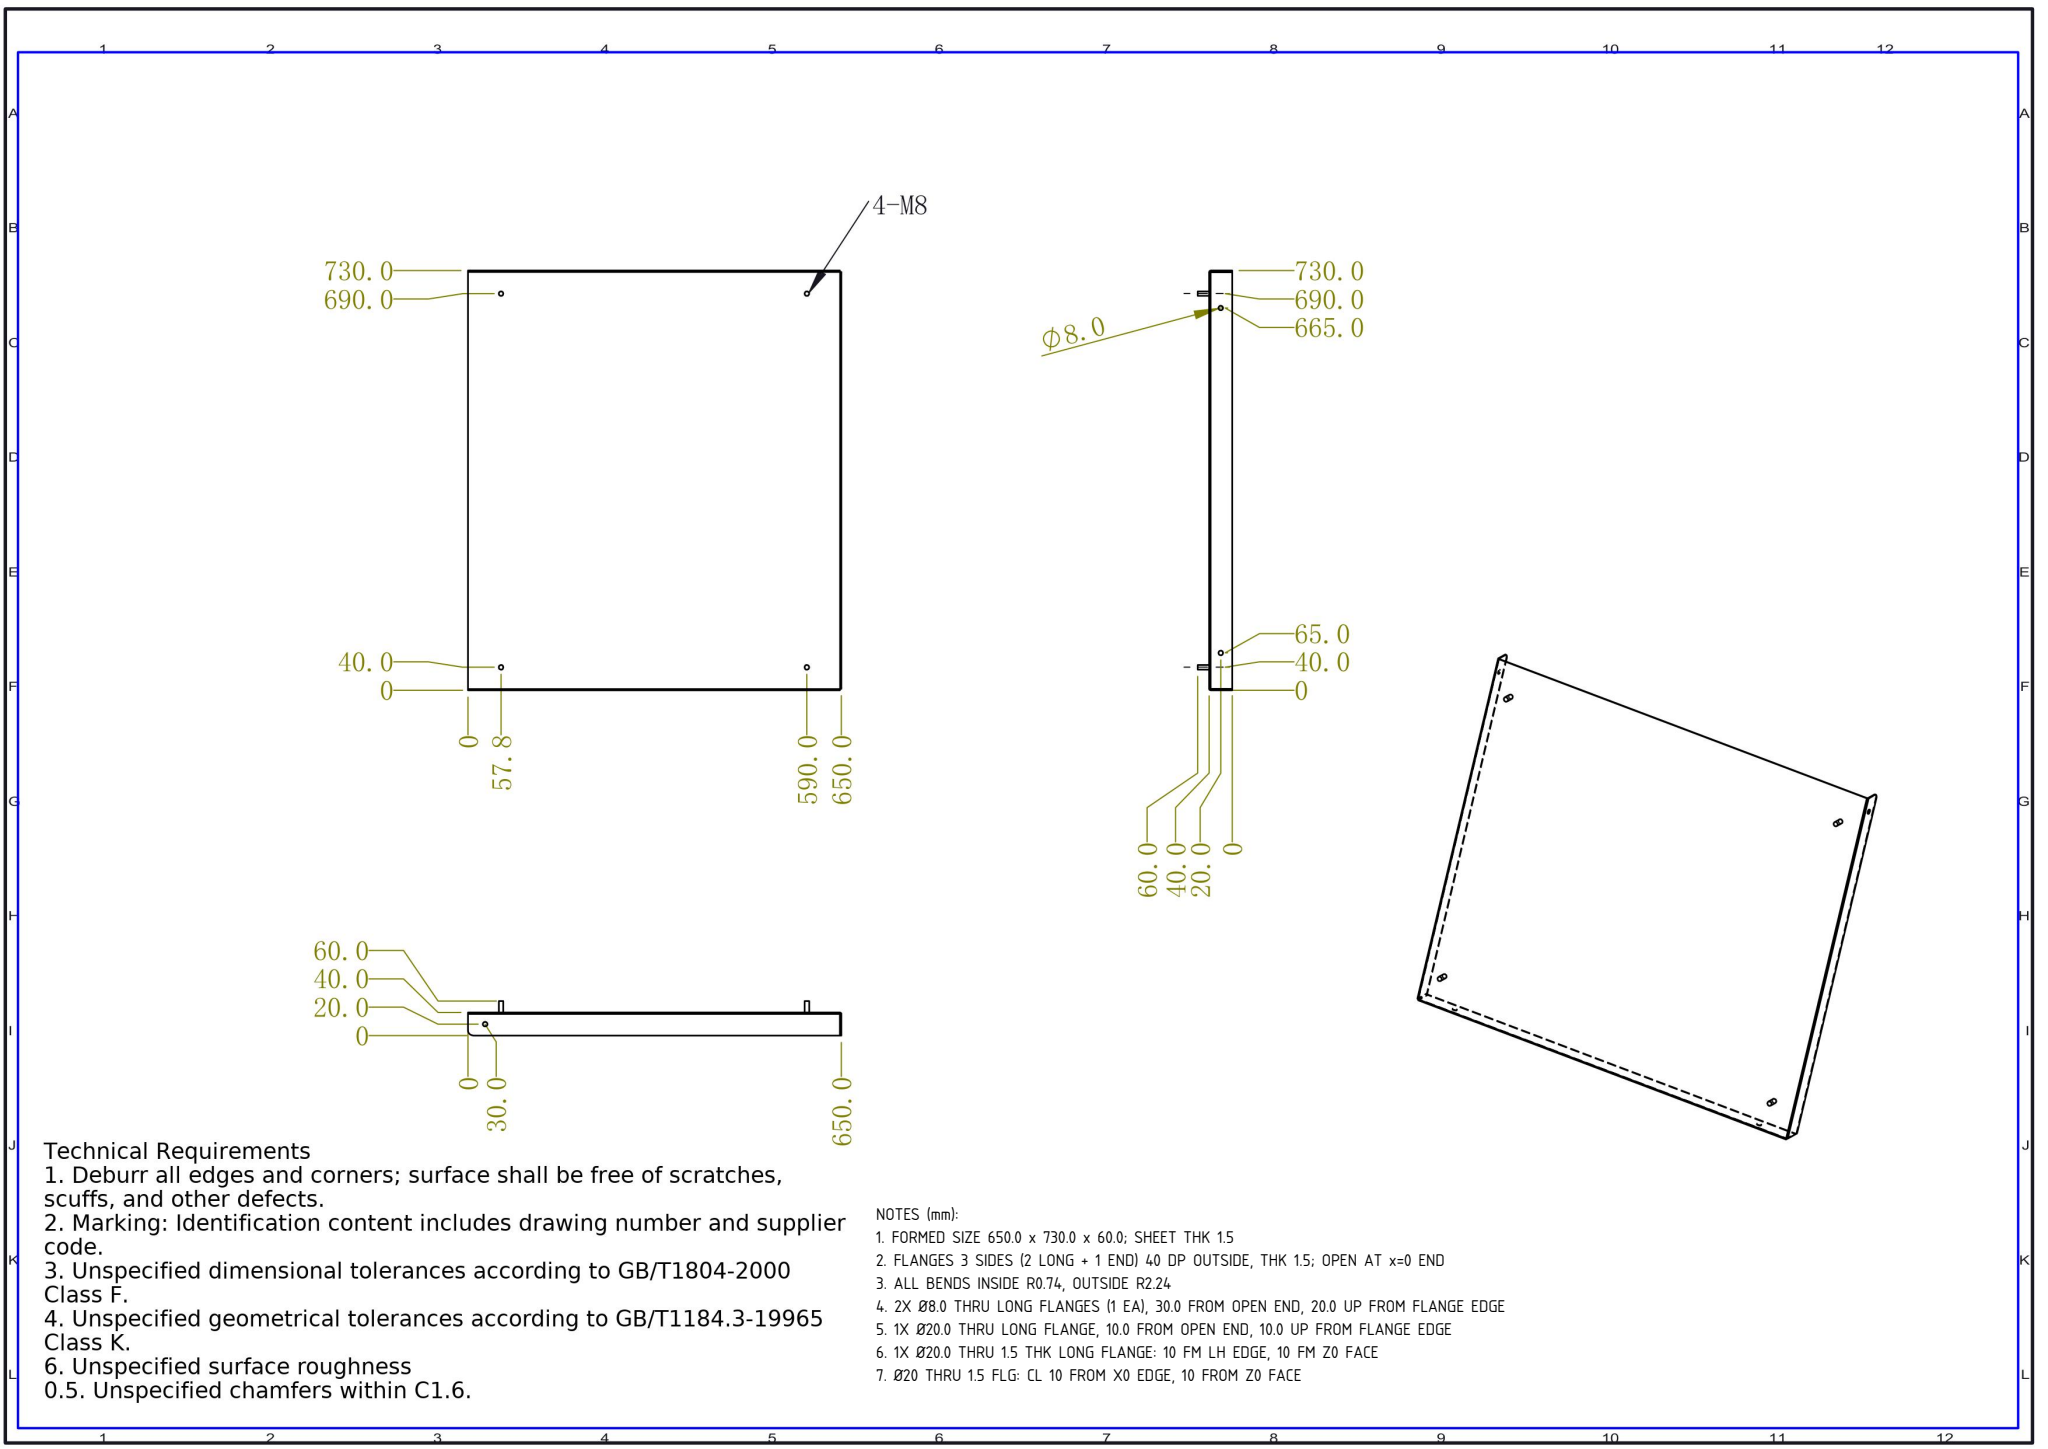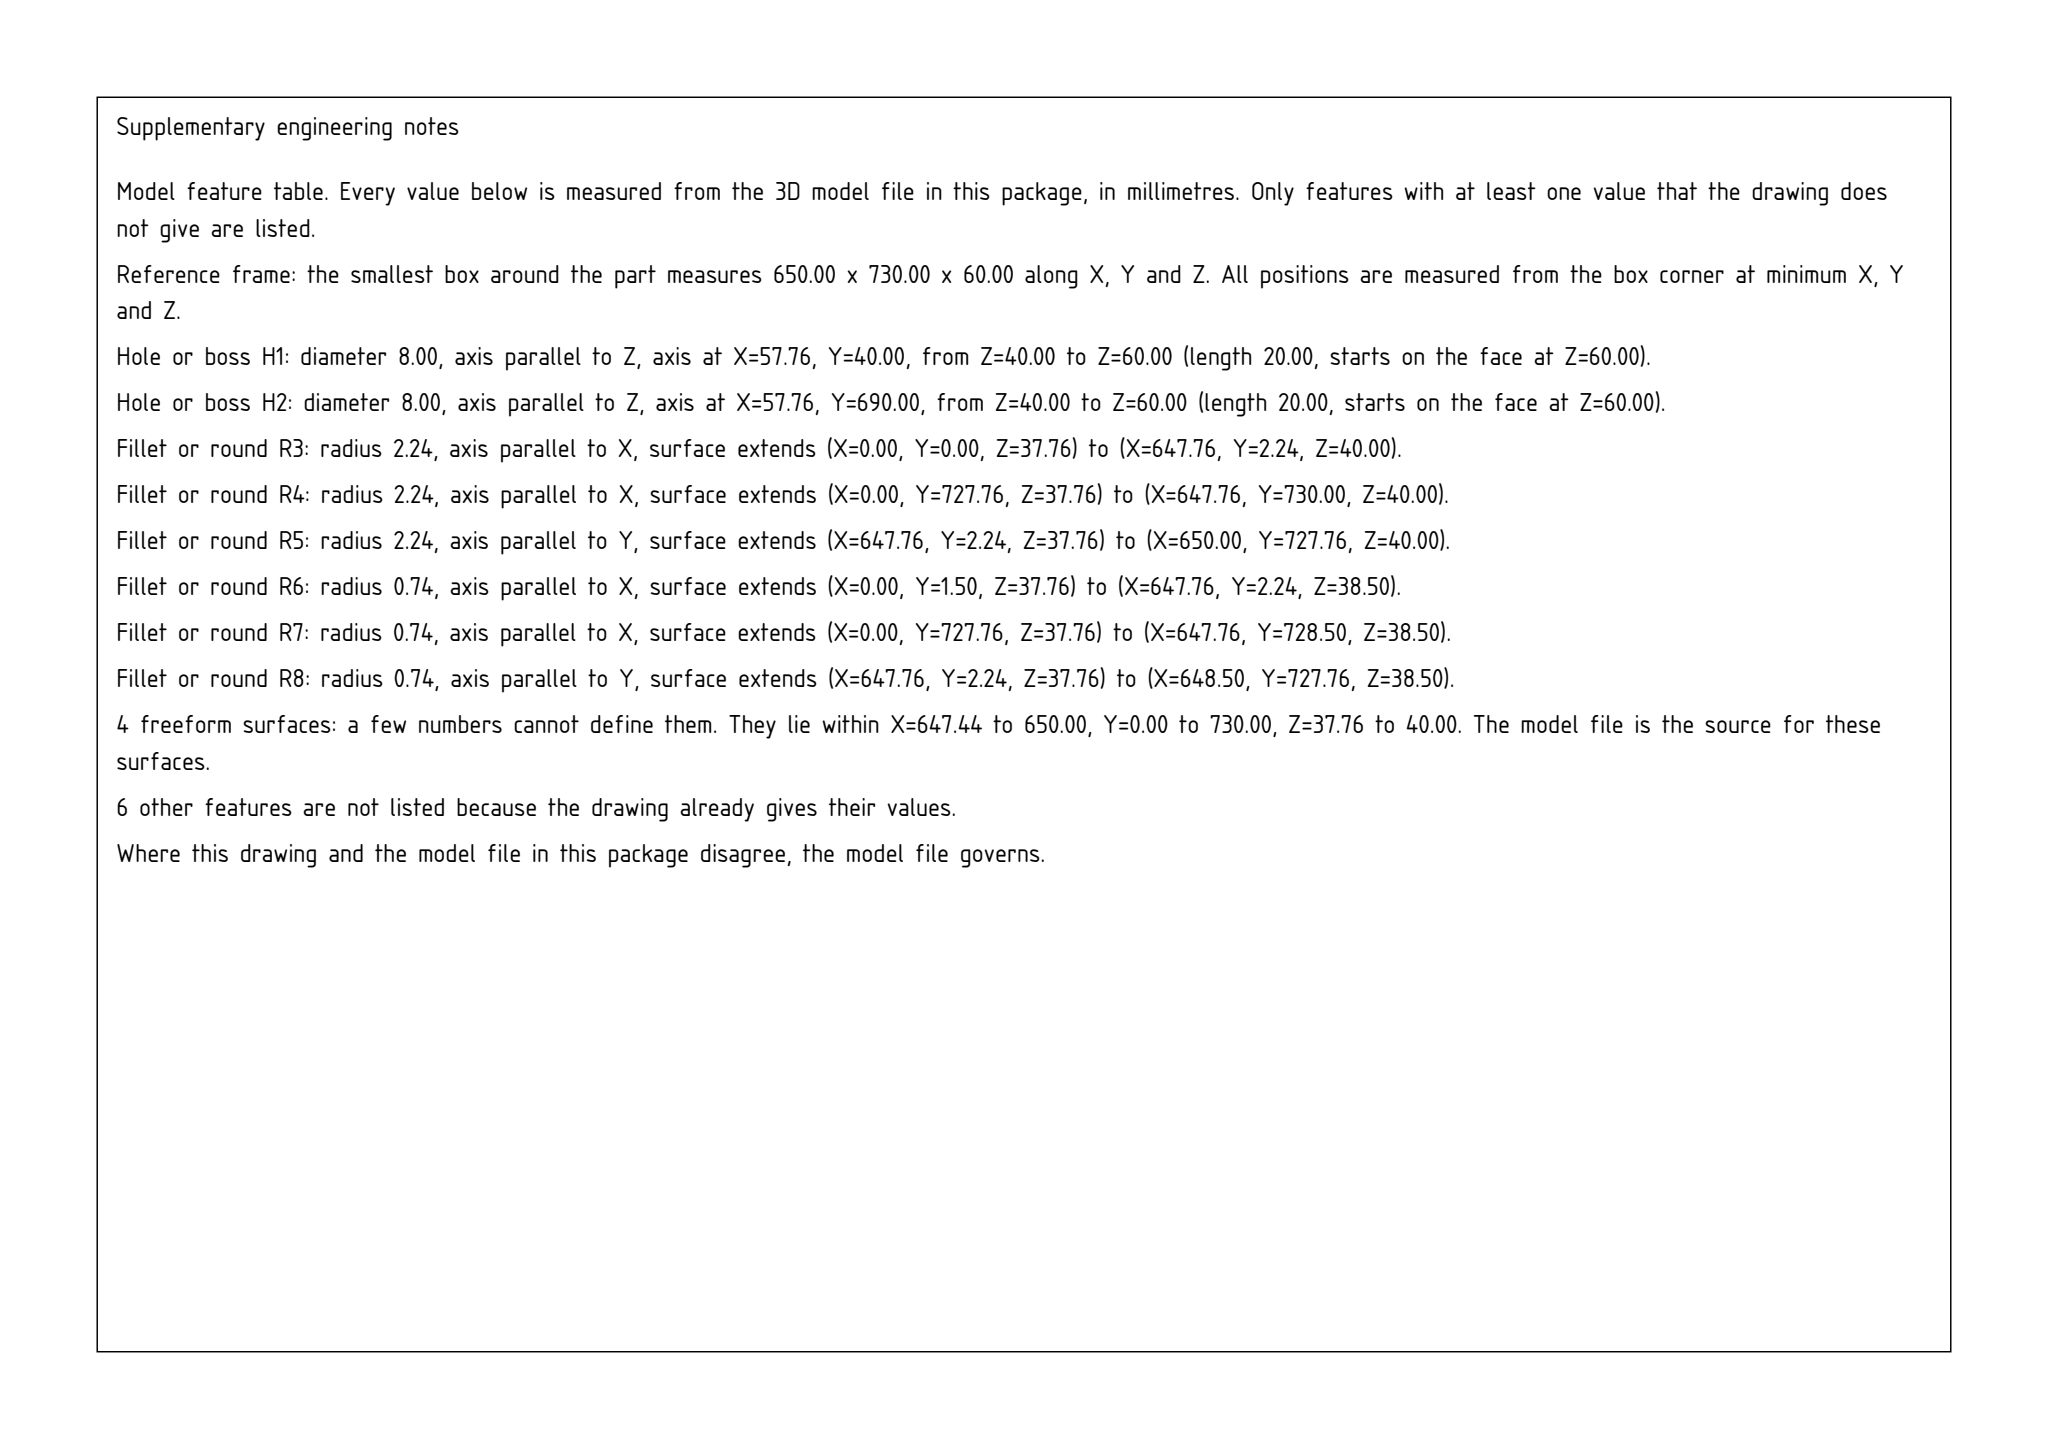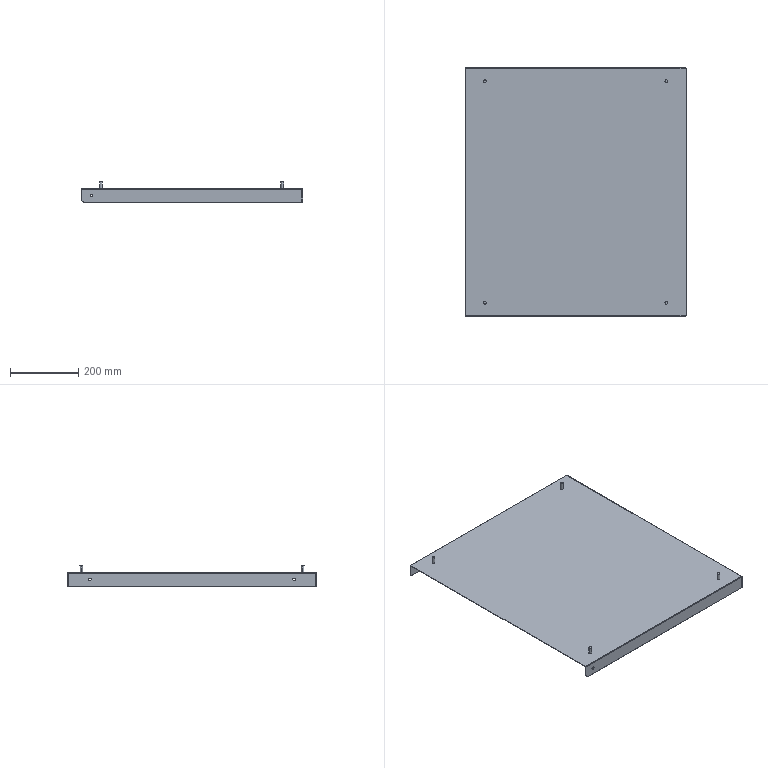Part | SolidWorks | mm | 1 solid | 52 faces | box 650 x 730 x 60 mm | volume 830096 mm3 | cylinder 24 | plane 24 | spline 4 | commonest cylinder face diameters 8 x16 4.473 x3 1.473 x3 20 x2
Drawing notes:
FORMED SIZE 650.0 x 730.0 x 60.0; SHEET THK 1.5 | from the solid: bbox 650.015 x 730.03 x 60.0; wall pairs z=38.5/40.0, y=0.02-1.52, x=648.5-650.0 give thk 1.5
FLANGES 3 SIDES (2 LONG + 1 END) 40 DP OUTSIDE, THK 1.5; OPEN AT x=0 END | from the solid: z planes 0/38.5/40.0; flange walls y=0.02-1.52, y=728.52-730.02, x=648.5-650.0; no wall at x=0
ALL BENDS INSIDE R0.74, OUTSIDE R2.24 | from the solid: bend cyls dia 1.473 (R0.74) & 4.473 (R2.24) about x @ y=2.25/727.78, about y @ x=647.76, z=37.76
2X Ø8.0 THRU LONG FLANGES (1 EA), 30.0 FROM OPEN END, 20.0 UP FROM FLANGE EDGE | from the solid: [8.0,"y",[30.0,null,20.0],1.5,4] = 2 holes thru 1.5 wall in both y-flanges
1X Ø20.0 THRU LONG FLANGE, 10.0 FROM OPEN END, 10.0 UP FROM FLANGE EDGE | from the solid: [20.0,"y",[10.0,null,10.0],1.5,2] thru 1.5 flange wall
1X Ø20.0 THRU 1.5 THK LONG FLANGE: 10 FM LH EDGE, 10 FM Z0 FACE | from the solid: cylinder [20.0,'y',[10.0,null,10.0],1.5] - axis parallel to Y, pierces a 1.5 thk long flange; X=10.0 from x=0 edge, Z=10.0 from z=0 face (bbox 650.015 x 730.03 x 60.0)
Ø20 THRU 1.5 FLG: CL 10 FROM X0 EDGE, 10 FROM Z0 FACE | from the solid: cylinders: [20.0,"y",[10.0,null,10.0],1.5,2] - Ø20 hole, axis along Y (thru 1.5 thk flange), centered x=10, z=10 from bbox min corner